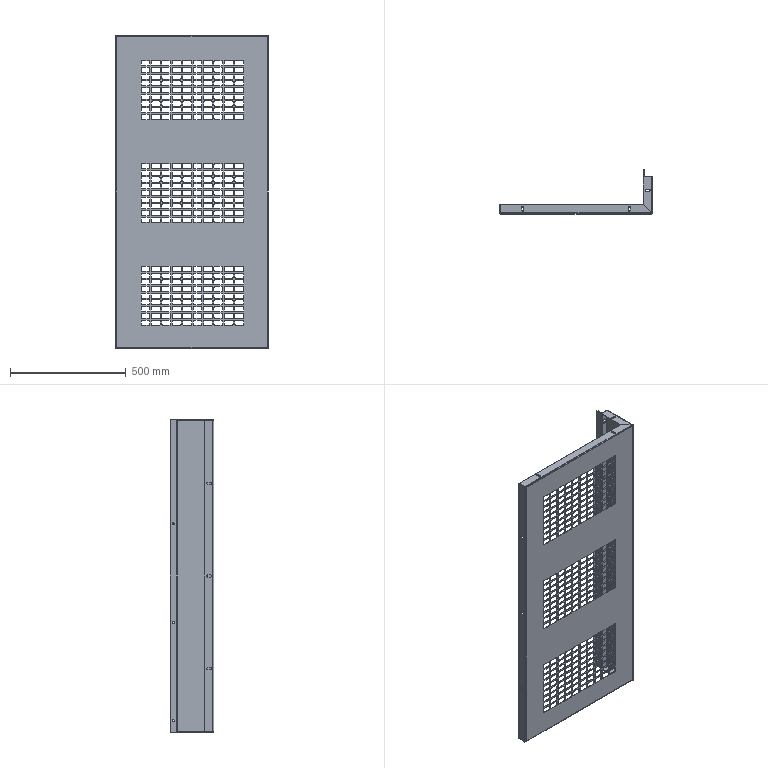Component | SolidWorks | RearLeftSidePlateAssembly-2_RearLeftSidePlate-1 | 1 solid | 2294 faces | volume 2129142 mm3 | plane 1156 | cylinder 1130 | spline 8 | commonest cylinder face diameters 6 x1080 10 x28 4 x8 8 x8 9 x6 | material Plain Carbon Steel